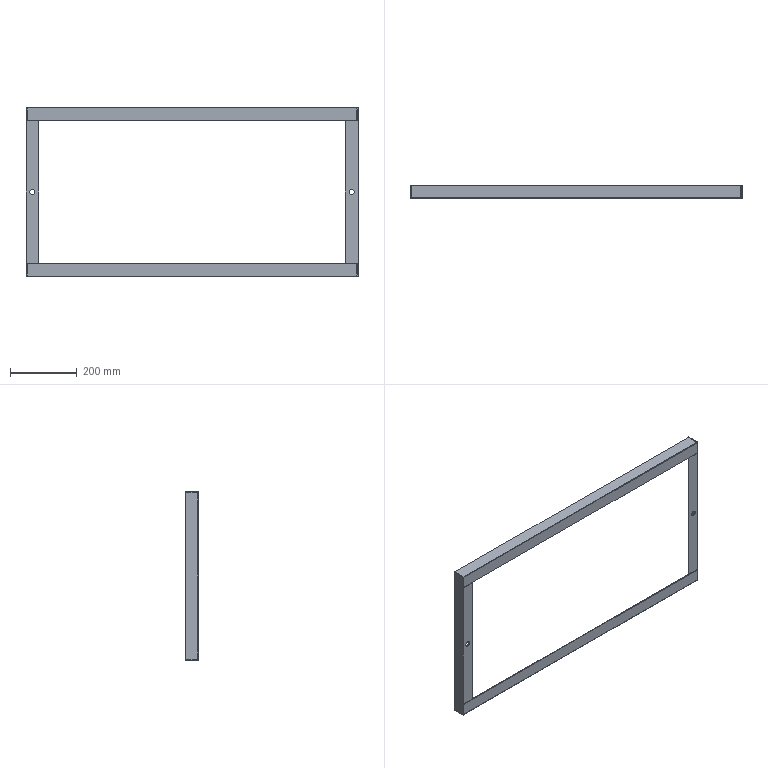Component | SolidWorks | AirFurnaceElectricalCabinet-AngleIronFrame-1 | 4 solids | 48 faces | box 997.6 x 38 x 507 mm | volume 637083 mm3 | plane 44 | cylinder 4 | commonest cylinder face diameters 16 x4
build123d program:
from build123d import *

# Parameters (mm, degrees)
EXTRUDE_THIN1_DEPTH = 495.5
EXTRUDE_THIN2_DEPTH = 253.5
EXTRUDE5_DEPTH      = 561.615
SKETCH5_R           = 8
CUT_EXTRUDE1_DEPTH  = 10
CHAMFER1_SIZE       = 1
CHAMFER2_SIZE       = 1
CHAMFER3_SIZE       = 1
CHAMFER4_SIZE       = 1


with BuildPart() as part:
    # Sketch1 → Extrude-Thin1 (new, symmetric)
    with BuildSketch(Plane(origin=(0, 0, 0), x_dir=(0, 0, -1), z_dir=(1, 0, 0))):
        Polygon((-253.5, 38), (-253.5, 0), (-215.5, 0), (-215.5, 3), (-250.5, 3), (-250.5, 38), align=None)
    extrude(amount=EXTRUDE_THIN1_DEPTH, both=True)


with BuildPart() as body_2:
    # Sketch2 → Extrude-Thin2 (new, symmetric)
    with BuildSketch(Plane.XY):
        Polygon((-498.8, 38), (-498.8, 0), (-460.8, 0), (-460.8, 3), (-495.8, 3), (-495.8, 38), align=None)
    extrude(amount=EXTRUDE_THIN2_DEPTH, both=True)

    # Sketch4 → Extrude5 (cut, symmetric)
    with BuildSketch(Plane(origin=(0, 3, 0), x_dir=(1, 0, 0), z_dir=(0, 1, 0))):
        Polygon((-495.8, -2555.684), (-495.8, -287.271), (-495.8, -213.5), (-303.611, -213.5), (1964.803, -213.5), (5092.776, -3499.621), (2632.174, -5841.805), align=None)
    extrude5 = extrude(amount=EXTRUDE5_DEPTH, both=True, mode=Mode.SUBTRACT)

    # Mirror1: Extrude5 across plane
    add(extrude5.mirror(Plane.XY), mode=Mode.SUBTRACT)


with BuildPart() as body_3:
    # Mirror2: mirrored copy
    add(part.part.mirror(Plane.XY))

    # Chamfer3
    chamfer3_edges = [body_3.edges().sort_by_distance(p)[0] for p in [
        (0, 0, -253.5),
    ]]
    chamfer(chamfer3_edges, length=CHAMFER3_SIZE)


with BuildPart() as body_4:
    # Mirror3: mirrored copy
    add(body_2.part.mirror(Plane(origin=(0, 0, 0), x_dir=(0, 0, 1), z_dir=(1, 0, 0))))


with BuildPart() as cut_extrude1_tool:
    # Sketch5 → Cut-Extrude1 (new, symmetric)
    with BuildSketch(Plane(origin=(0, 0, 0), x_dir=(1, 0, 0), z_dir=(0, 1, 0))):
        with Locations(Location((479.8, 0, 0), (0, 0, 270))):
            Circle(SKETCH5_R)
        with Locations(Location((-479.8, 0, 0), (0, 0, 270))):
            Circle(SKETCH5_R)
    extrude(amount=CUT_EXTRUDE1_DEPTH, both=True)


with BuildPart() as body_2_1:
    add(body_2.part)

    # Cut-Extrude1: cut by cut_extrude1_tool
    add(cut_extrude1_tool.part, mode=Mode.SUBTRACT)

    # Chamfer4
    chamfer4_edges = [body_2_1.edges().sort_by_distance(p)[0] for p in [
        (-497.3, 0, 253.5),
        (-498.8, 19, -253.5),
        (-497.3, 0, -253.5),
    ]]
    chamfer(chamfer4_edges, length=CHAMFER4_SIZE)


with BuildPart() as body_4_1:
    add(body_4.part)

    # Cut-Extrude1: cut by cut_extrude1_tool
    add(cut_extrude1_tool.part, mode=Mode.SUBTRACT)

    # Chamfer2
    chamfer2_edges = [body_4_1.edges().sort_by_distance(p)[0] for p in [
        (497.3, 0, 253.5),
        (498.8, 19, -253.5),
        (497.3, 0, -253.5),
    ]]
    chamfer(chamfer2_edges, length=CHAMFER2_SIZE)


with BuildPart() as part_1:
    add(part.part)

    # Chamfer1
    chamfer1_edges = [part_1.edges().sort_by_distance(p)[0] for p in [
        (0, 0, 253.5),
    ]]
    chamfer(chamfer1_edges, length=CHAMFER1_SIZE)


solid = Compound([body_3.part, body_2_1.part, body_4_1.part, part_1.part])